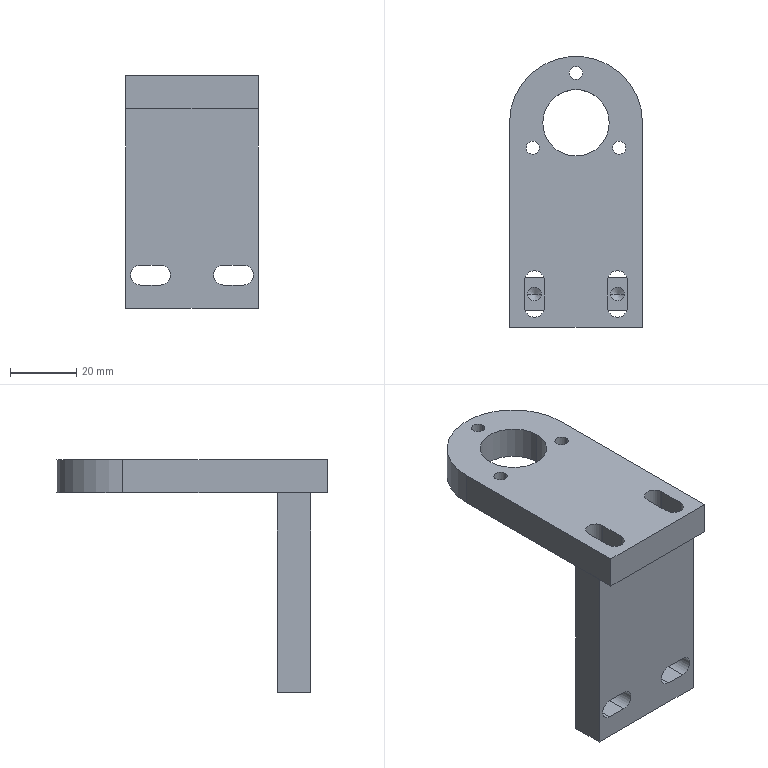Component | SolidWorks | EncoderMountingSeat-1 | 2 solids | 53 faces | box 40 x 81.5 x 70 mm | volume 47965 mm3 | cylinder 27 | plane 22 | cone 4 | commonest cylinder face diameters 6 x8 7 x6 4 x6 4.2 x4 20 x2 40 x1
build123d program:
from build123d import *

# Parameters (mm, degrees)
SKETCH1_R                  = 10
BOSS_EXTRUDE1_DEPTH        = 10
SKETCH3_R                  = 2
CUT_EXTRUDE1_DEPTH         = 92.336
SKETCH4_R                  = 3.5
CUT_EXTRUDE2_DEPTH         = 3
SKETCH5_W                  = 40
SKETCH5_H                  = 10
BOSS_EXTRUDE3_DEPTH        = 60
M5_TAPPED_HOLE1_AT_2_COUNT = 2
M5_TAPPED_HOLE1_AT_2_PITCH = 25
CUT_EXTRUDE3_DEPTH         = 10
CUT_EXTRUDE4_DEPTH         = 70


with BuildPart() as part:
    # Sketch1 → Boss-Extrude1 (new body)
    with BuildSketch(Plane.XY):
        with BuildLine():
            Line((0, 0), (0, 61.5))
            ThreePointArc((0, 61.5), (20, 81.5), (40, 61.5))
            Line((40, 61.5), (40, 0))
            Line((40, 0), (0, 0))
        make_face()
        with Locations((20, 61.5)):
            Circle(SKETCH1_R, mode=Mode.SUBTRACT)
    extrude(amount=BOSS_EXTRUDE1_DEPTH)

    # Sketch3 → Cut-Extrude1 (cut, through all)
    with BuildSketch(Plane.XY.offset(10)):
        with Locations((20, 76.5)):
            Circle(SKETCH3_R)
        with Locations((7.01, 54)):
            Circle(SKETCH3_R)
        with Locations((32.99, 54)):
            Circle(SKETCH3_R)
    extrude(amount=-CUT_EXTRUDE1_DEPTH, mode=Mode.SUBTRACT)

    # Sketch4 → Cut-Extrude2 (cut)
    with BuildSketch(Plane.XY.offset(10)):
        with Locations((20, 76.5)):
            Circle(SKETCH4_R)
        with Locations((7.01, 54)):
            Circle(SKETCH4_R)
        with Locations((32.99, 54)):
            Circle(SKETCH4_R)
    extrude(amount=-CUT_EXTRUDE2_DEPTH, mode=Mode.SUBTRACT)

    # Sketch8 → Cut-Extrude3 (cut)
    with BuildSketch(Plane(origin=(0, 0, 0), x_dir=(-1, 0, 0), z_dir=(0, 0, -1))):
        with BuildLine():
            Line((-29.5, 14), (-29.5, 6))
            ThreePointArc((-29.5, 6), (-32.5, 3), (-35.5, 6))
            Line((-35.5, 6), (-35.5, 14))
            ThreePointArc((-35.5, 14), (-32.5, 17), (-29.5, 14))
        make_face()
        with BuildLine():
            Line((-4.5, 14), (-4.5, 6))
            ThreePointArc((-4.5, 6), (-7.5, 3), (-10.5, 6))
            Line((-10.5, 6), (-10.5, 14))
            ThreePointArc((-10.5, 14), (-7.5, 17), (-4.5, 14))
        make_face()
    extrude(amount=-CUT_EXTRUDE3_DEPTH, mode=Mode.SUBTRACT)


with BuildPart() as body_2:
    # Sketch5 → Boss-Extrude3 (new body)
    with BuildSketch(Plane.XY.offset(10)):
        with Locations((20, 10)):
            Rectangle(SKETCH5_W, SKETCH5_H)
    extrude(amount=BOSS_EXTRUDE3_DEPTH)

    # Sketch7 → M5 Tapped Hole1 (revolve, cut)
    with BuildSketch(Plane(origin=(7.5, 10, 10), x_dir=(0, 1, 0), z_dir=(1, 0, 0))):
        Polygon((0, 0), (0, 13.662), (2.1, 12.4), (2.1, 0), align=None)
    m5_tapped_hole1 = revolve(axis=Axis((7.5, 10, 3.65), (0, 0, 1)), mode=Mode.SUBTRACT)

    # M5 Tapped Hole1 at 2: M5 Tapped Hole1 ×2
    with Locations(*[(i * M5_TAPPED_HOLE1_AT_2_PITCH, 0, 0) for i in range(1, M5_TAPPED_HOLE1_AT_2_COUNT)]):
        add(m5_tapped_hole1, mode=Mode.SUBTRACT)

    # Sketch9 → Cut-Extrude4 (cut)
    with BuildSketch(Plane.XZ.offset(-5)):
        with BuildLine():
            Line((4.5, 63), (10.5, 63))
            ThreePointArc((10.5, 63), (13.5, 60), (10.5, 57))
            Line((10.5, 57), (4.5, 57))
            ThreePointArc((4.5, 57), (1.5, 60), (4.5, 63))
        make_face()
        with BuildLine():
            Line((29.5, 63), (35.5, 63))
            ThreePointArc((35.5, 63), (38.5, 60), (35.5, 57))
            Line((35.5, 57), (29.5, 57))
            ThreePointArc((29.5, 57), (26.5, 60), (29.5, 63))
        make_face()
    extrude(amount=-CUT_EXTRUDE4_DEPTH, mode=Mode.SUBTRACT)


solid = Compound([part.part, body_2.part])

# Placed as in the assembly
solid = solid.moved(Location((-279.507, -259.411, 690), (-180, 0, 180)))